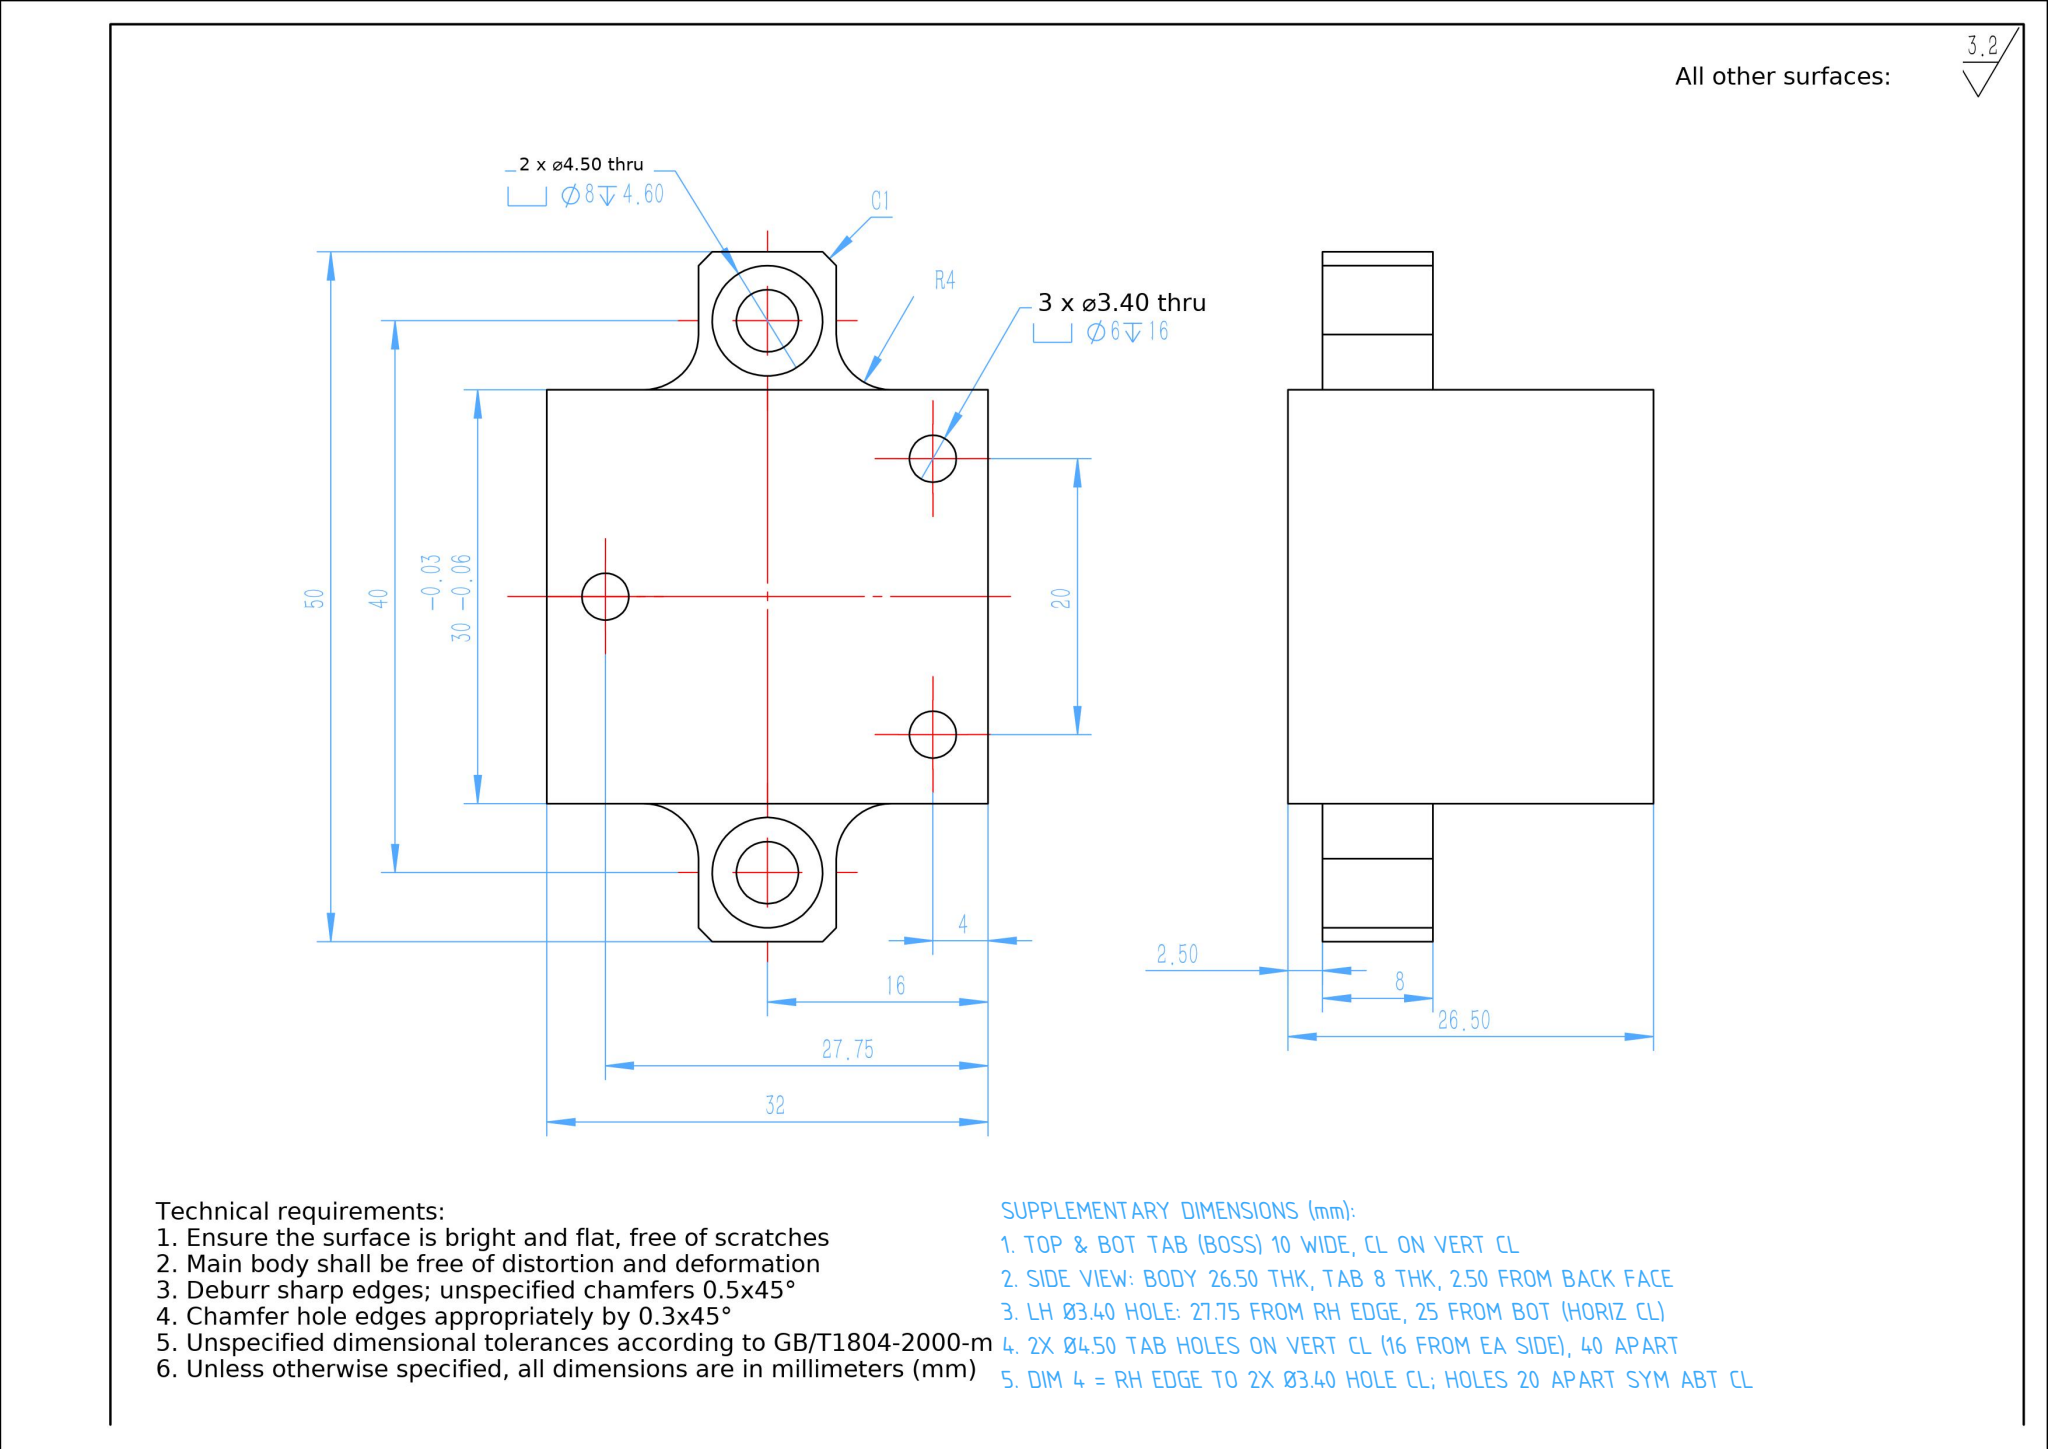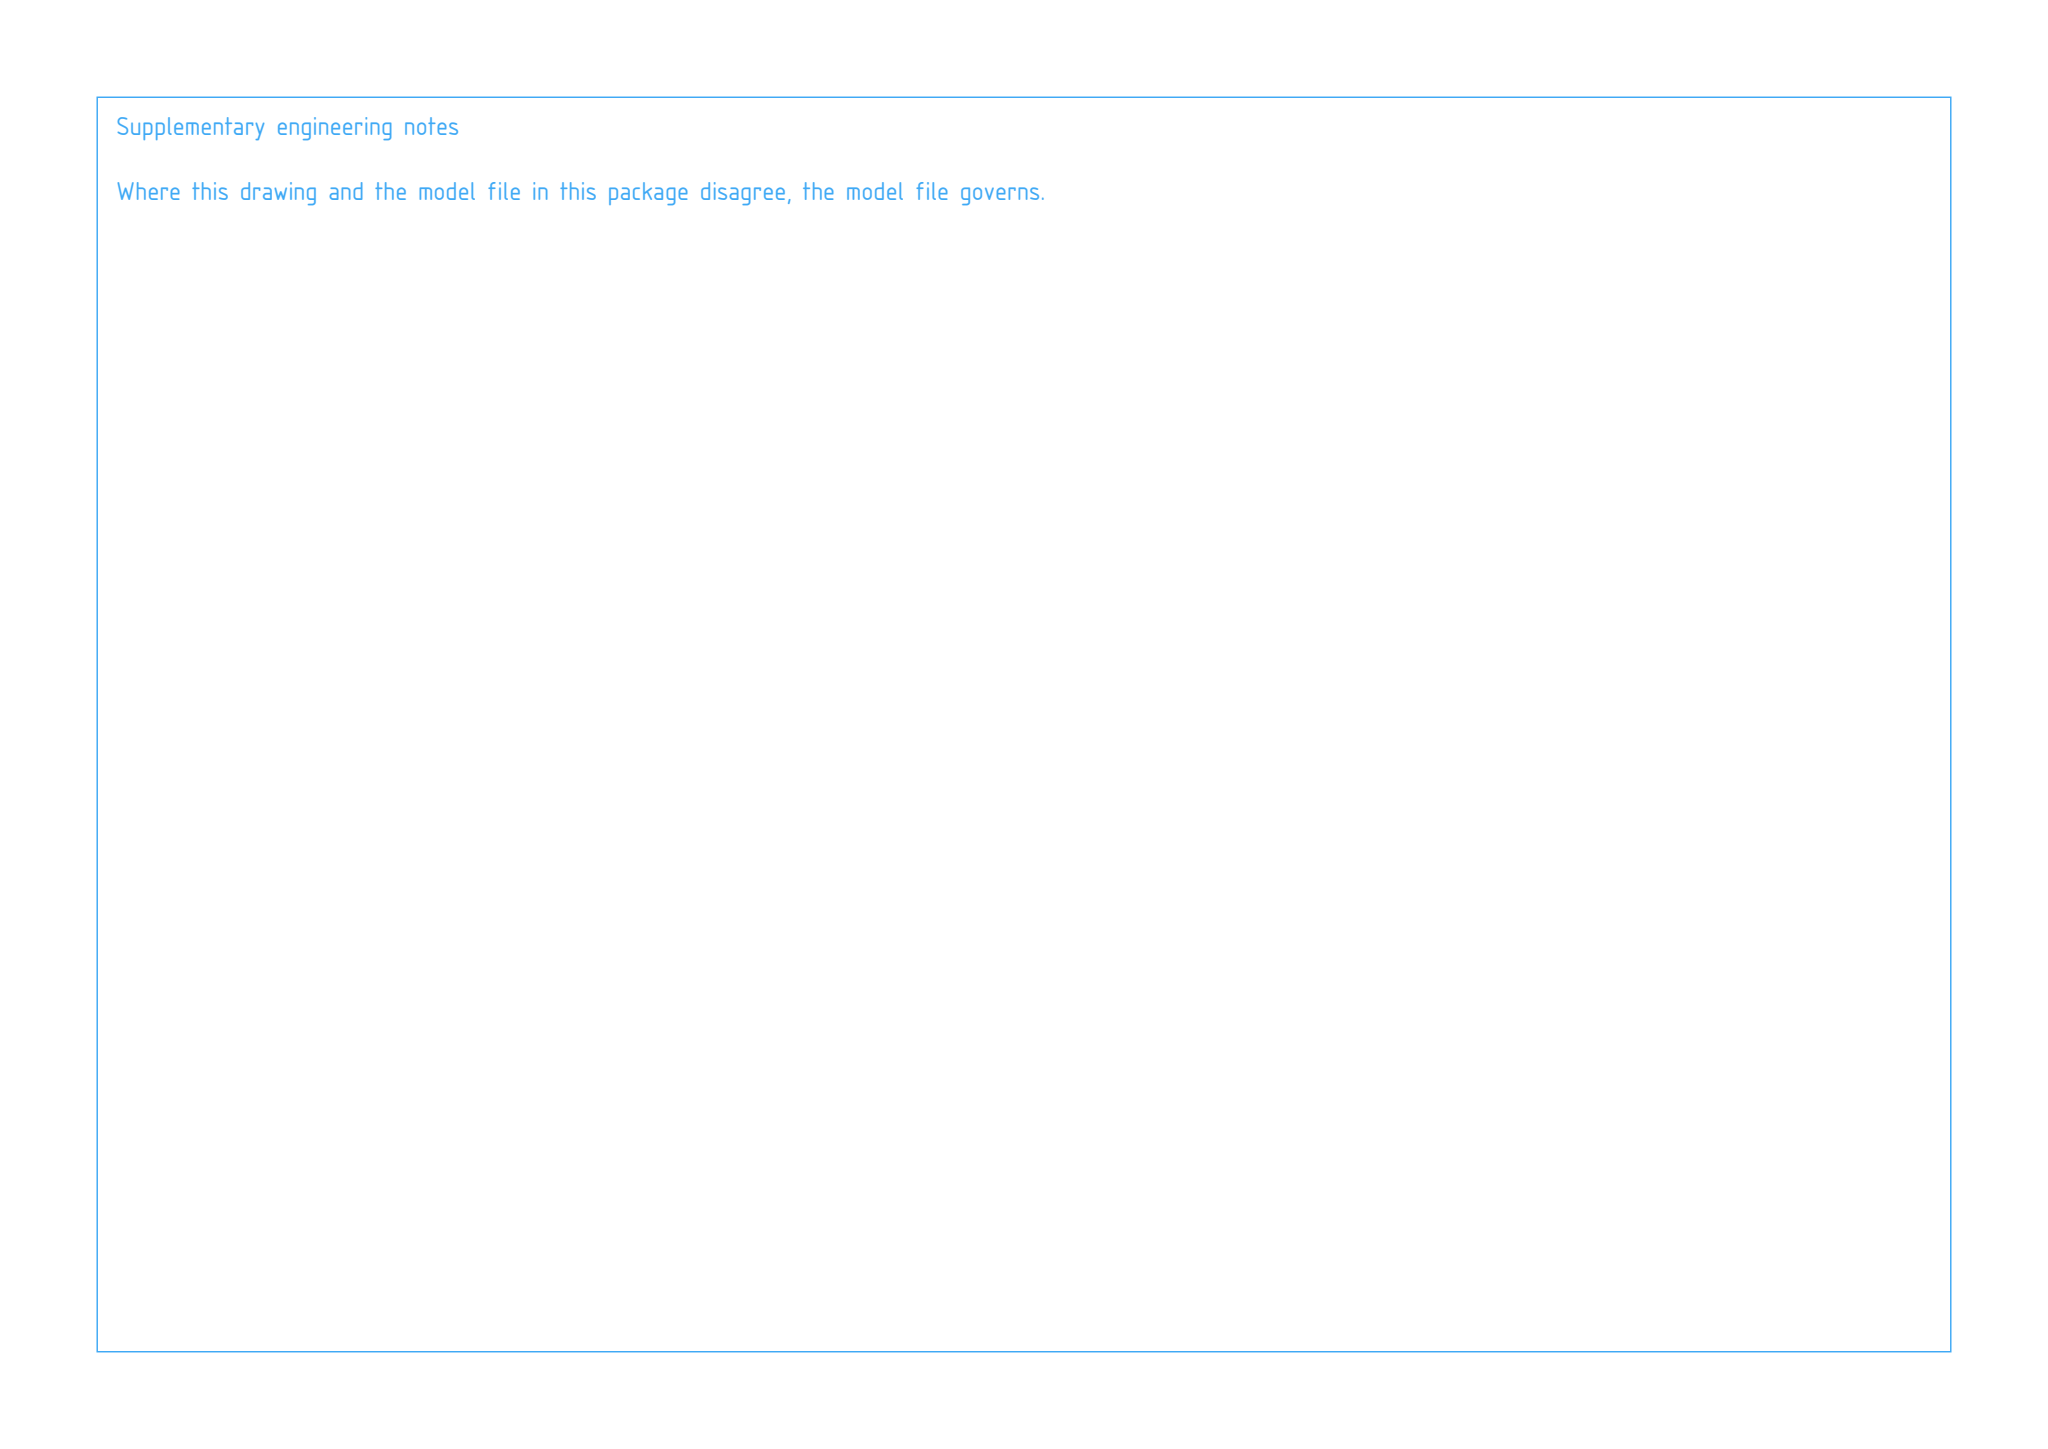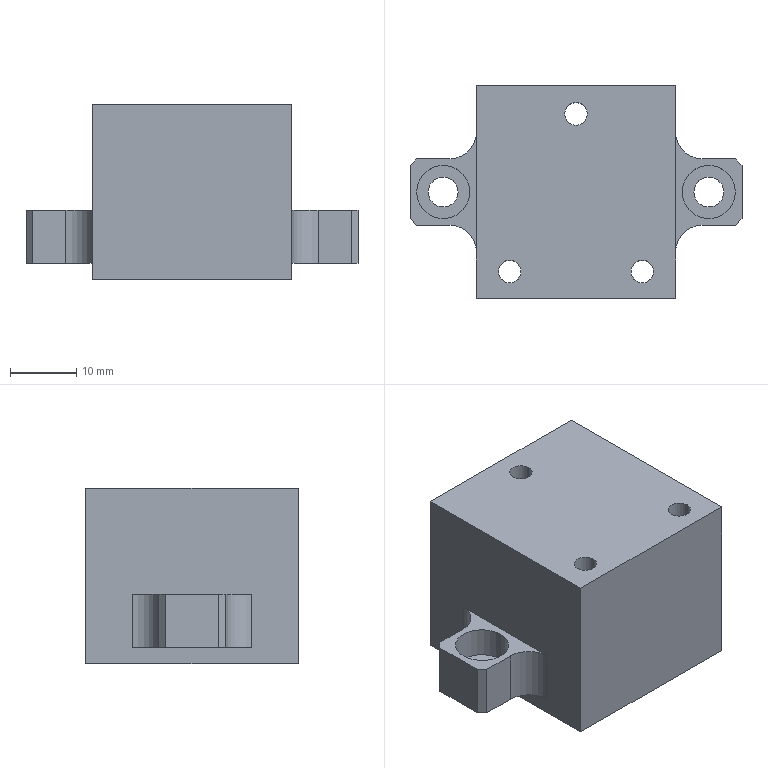Part | SolidWorks | mm | 1 solid | 49 faces | box 50 x 32 x 26.5 mm | volume 24920 mm3 | plane 25 | cylinder 24 | commonest cylinder face diameters 8 x8 6 x6 3.4 x6 4.5 x4
build123d program:
from build123d import *

# Parameters (mm, degrees)
SKETCH1_W                                         = 30
SKETCH1_H                                         = 32
BOSS_EXTRUDE1_DEPTH                               = 26.5
SKETCH2_W                                         = 50
SKETCH2_H                                         = 10
BOSS_EXTRUDE2_DEPTH                               = 8
FILLET1_R                                         = 4
CHAMFER1_SIZE                                     = 1
HOLE_SIZE_ACCORDING_TO_HEXAGON_SOCKET_D           = 4.5
HOLE_SIZE_ACCORDING_TO_HEXAGON_SOCKET_CBORE_D     = 8
HOLE_SIZE_ACCORDING_TO_HEXAGON_SOCKET_CBORE_DEPTH = 4.6
HOLE_SIZE_ACCORDING_TO_HEXAGON_SO_2_D             = 3.4
HOLE_SIZE_ACCORDING_TO_HEXAGON_SO_2_CBORE_D       = 6
HOLE_SIZE_ACCORDING_TO_HEXAGON_SO_2_CBORE_DEPTH   = 16


with BuildPart() as part:
    # Sketch1 → Boss-Extrude1 (new body)
    with BuildSketch(Plane.XY):
        Rectangle(SKETCH1_W, SKETCH1_H)
    extrude(amount=-BOSS_EXTRUDE1_DEPTH)

    # Sketch2 → Boss-Extrude2 (add)
    with BuildSketch(Plane(origin=(0, 0, -24), x_dir=(-1, 0, 0), z_dir=(0, 0, -1))):
        Rectangle(SKETCH2_W, SKETCH2_H)
    extrude(amount=-BOSS_EXTRUDE2_DEPTH)

    # Fillet1
    fillet1_edges = [part.edges().sort_by_distance(p)[0] for p in [
        (-15, 5, -20),
        (-15, -5, -20),
        (15, -5, -20),
        (15, 5, -20),
    ]]
    fillet(fillet1_edges, radius=FILLET1_R)

    # Chamfer1
    chamfer1_edges = [part.edges().sort_by_distance(p)[0] for p in [
        (25, 5, -20),
        (-25, 5, -20),
        (-25, -5, -20),
        (25, -5, -20),
    ]]
    chamfer(chamfer1_edges, length=CHAMFER1_SIZE)

    # Hole Size _ according to_ Hexagon Socket (through all)
    with Locations(Plane.XY.offset(-16)):
        with Locations((-20, 0), (20, 0)):
            CounterBoreHole(HOLE_SIZE_ACCORDING_TO_HEXAGON_SOCKET_D / 2, HOLE_SIZE_ACCORDING_TO_HEXAGON_SOCKET_CBORE_D / 2, HOLE_SIZE_ACCORDING_TO_HEXAGON_SOCKET_CBORE_DEPTH)

    # Hole Size _ according to_ Hexagon So 2 (through all)
    with Locations(Plane(origin=(0, 0, -26.5), x_dir=(-1, 0, 0), z_dir=(0, 0, -1))):
        with Locations((0, 11.75), (-10, -12), (10, -12)):
            CounterBoreHole(HOLE_SIZE_ACCORDING_TO_HEXAGON_SO_2_D / 2, HOLE_SIZE_ACCORDING_TO_HEXAGON_SO_2_CBORE_D / 2, HOLE_SIZE_ACCORDING_TO_HEXAGON_SO_2_CBORE_DEPTH)


solid = part.part